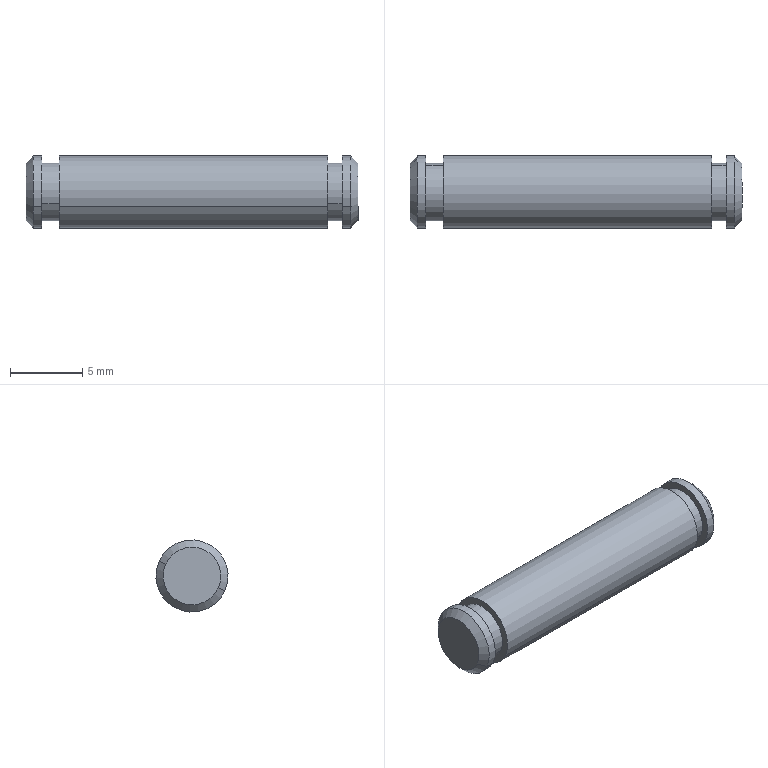Component | SolidWorks | LeverHydraulicRod22-1_HLKA-22_-2-1 | 1 solid | 20 faces | box 23 x 5 x 5 mm | volume 432 mm3 | cylinder 10 | plane 6 | cone 4 | commonest cylinder face diameters 5 x6 4 x4
STEP:
#1=CARTESIAN_POINT('',(-3.072,4.4,-3.091));
#2=VERTEX_POINT('',#1);
#3=CARTESIAN_POINT('',(-3.072,4.58,-3.011));
#4=VERTEX_POINT('',#3);
#5=CARTESIAN_POINT('',(-3.072,4.49,-3.051));
#6=DIRECTION('',(1.,0.,0.));
#7=DIRECTION('',(0.,0.9136,0.4066));
#8=AXIS2_PLACEMENT_3D('',#5,#6,#7);
#9=CIRCLE('',#8,0.09843);
#10=EDGE_CURVE('',#2,#4,#9,.T.);
#11=ORIENTED_EDGE('',*,*,#10,.F.);
#12=CARTESIAN_POINT('',(-3.095,4.4,-3.091));
#13=VERTEX_POINT('',#12);
#14=CARTESIAN_POINT('',(-2.209,4.4,-3.091));
#15=DIRECTION('',(-1.,-0.,-0.));
#16=VECTOR('',#15,39.37);
#17=LINE('',#14,#16);
#18=EDGE_CURVE('',#2,#13,#17,.T.);
#19=ORIENTED_EDGE('',*,*,#18,.T.);
#20=CARTESIAN_POINT('',(-3.095,4.58,-3.011));
#21=VERTEX_POINT('',#20);
#22=CARTESIAN_POINT('',(-3.095,4.49,-3.051));
#23=DIRECTION('',(1.,0.,0.));
#24=DIRECTION('',(0.,-0.9136,-0.4066));
#25=AXIS2_PLACEMENT_3D('',#22,#23,#24);
#26=CIRCLE('',#25,0.09843);
#27=EDGE_CURVE('',#13,#21,#26,.T.);
#28=ORIENTED_EDGE('',*,*,#27,.T.);
#29=CARTESIAN_POINT('',(-2.209,4.58,-3.011));
#30=DIRECTION('',(-1.,-0.,-0.));
#31=VECTOR('',#30,39.37);
#32=LINE('',#29,#31);
#33=EDGE_CURVE('',#4,#21,#32,.T.);
#34=ORIENTED_EDGE('',*,*,#33,.F.);
#35=EDGE_LOOP('',(#11,#19,#28,#34));
#36=FACE_OUTER_BOUND('',#35,.T.);
#37=CARTESIAN_POINT('',(-2.209,4.49,-3.051));
#38=DIRECTION('',(-1.,-0.,-0.));
#39=DIRECTION('',(0.,0.9136,0.4066));
#40=AXIS2_PLACEMENT_3D('',#37,#38,#39);
#41=CYLINDRICAL_SURFACE('',#40,0.09843);
#42=ADVANCED_FACE('',(#36),#41,.T.);
#43=CARTESIAN_POINT('',(-3.115,4.562,-3.019));
#44=VERTEX_POINT('',#43);
#45=CARTESIAN_POINT('',(-3.115,4.418,-3.083));
#46=VERTEX_POINT('',#45);
#47=CARTESIAN_POINT('',(-3.115,4.49,-3.051));
#48=DIRECTION('',(-1.,-0.,-0.));
#49=DIRECTION('',(0.,-0.9136,-0.4066));
#50=AXIS2_PLACEMENT_3D('',#47,#48,#49);
#51=CIRCLE('',#50,0.07874);
#52=EDGE_CURVE('',#44,#46,#51,.T.);
#53=ORIENTED_EDGE('',*,*,#52,.F.);
#54=CARTESIAN_POINT('',(-3.095,4.58,-3.011));
#55=DIRECTION('',(0.7071,0.646,0.2875));
#56=VECTOR('',#55,39.37);
#57=LINE('',#54,#56);
#58=EDGE_CURVE('',#44,#21,#57,.T.);
#59=ORIENTED_EDGE('',*,*,#58,.T.);
#60=ORIENTED_EDGE('',*,*,#27,.F.);
#61=CARTESIAN_POINT('',(-3.095,4.4,-3.091));
#62=DIRECTION('',(0.7071,-0.646,-0.2875));
#63=VECTOR('',#62,39.37);
#64=LINE('',#61,#63);
#65=EDGE_CURVE('',#46,#13,#64,.T.);
#66=ORIENTED_EDGE('',*,*,#65,.F.);
#67=EDGE_LOOP('',(#53,#59,#60,#66));
#68=FACE_OUTER_BOUND('',#67,.T.);
#69=CARTESIAN_POINT('',(-3.095,4.49,-3.051));
#70=DIRECTION('',(1.,0.,0.));
#71=DIRECTION('',(0.,-0.9136,-0.4066));
#72=AXIS2_PLACEMENT_3D('',#69,#70,#71);
#73=CONICAL_SURFACE('',#72,0.09843,0.7854);
#74=ADVANCED_FACE('',(#68),#73,.T.);
#75=CARTESIAN_POINT('',(-2.229,4.58,-3.011));
#76=VERTEX_POINT('',#75);
#77=CARTESIAN_POINT('',(-2.229,4.4,-3.091));
#78=VERTEX_POINT('',#77);
#79=CARTESIAN_POINT('',(-2.229,4.49,-3.051));
#80=DIRECTION('',(-1.,-0.,-0.));
#81=DIRECTION('',(0.,-0.9136,-0.4066));
#82=AXIS2_PLACEMENT_3D('',#79,#80,#81);
#83=CIRCLE('',#82,0.09843);
#84=EDGE_CURVE('',#76,#78,#83,.T.);
#85=ORIENTED_EDGE('',*,*,#84,.T.);
#86=CARTESIAN_POINT('',(-2.253,4.4,-3.091));
#87=VERTEX_POINT('',#86);
#88=CARTESIAN_POINT('',(-2.209,4.4,-3.091));
#89=DIRECTION('',(-1.,-0.,-0.));
#90=VECTOR('',#89,39.37);
#91=LINE('',#88,#90);
#92=EDGE_CURVE('',#78,#87,#91,.T.);
#93=ORIENTED_EDGE('',*,*,#92,.T.);
#94=CARTESIAN_POINT('',(-2.253,4.58,-3.011));
#95=VERTEX_POINT('',#94);
#96=CARTESIAN_POINT('',(-2.253,4.49,-3.051));
#97=DIRECTION('',(1.,0.,0.));
#98=DIRECTION('',(0.,-0.9136,-0.4066));
#99=AXIS2_PLACEMENT_3D('',#96,#97,#98);
#100=CIRCLE('',#99,0.09843);
#101=EDGE_CURVE('',#87,#95,#100,.T.);
#102=ORIENTED_EDGE('',*,*,#101,.T.);
#103=CARTESIAN_POINT('',(-2.209,4.58,-3.011));
#104=DIRECTION('',(-1.,-0.,-0.));
#105=VECTOR('',#104,39.37);
#106=LINE('',#103,#105);
#107=EDGE_CURVE('',#76,#95,#106,.T.);
#108=ORIENTED_EDGE('',*,*,#107,.F.);
#109=EDGE_LOOP('',(#85,#93,#102,#108));
#110=FACE_OUTER_BOUND('',#109,.T.);
#111=CARTESIAN_POINT('',(-2.209,4.49,-3.051));
#112=DIRECTION('',(-1.,-0.,-0.));
#113=DIRECTION('',(0.,0.9136,0.4066));
#114=AXIS2_PLACEMENT_3D('',#111,#112,#113);
#115=CYLINDRICAL_SURFACE('',#114,0.09843);
#116=ADVANCED_FACE('',(#110),#115,.T.);
#117=CARTESIAN_POINT('',(-2.209,4.418,-3.083));
#118=VERTEX_POINT('',#117);
#119=CARTESIAN_POINT('',(-2.209,4.562,-3.019));
#120=VERTEX_POINT('',#119);
#121=CARTESIAN_POINT('',(-2.209,4.49,-3.051));
#122=DIRECTION('',(1.,0.,0.));
#123=DIRECTION('',(0.,-0.9136,-0.4066));
#124=AXIS2_PLACEMENT_3D('',#121,#122,#123);
#125=CIRCLE('',#124,0.07874);
#126=EDGE_CURVE('',#118,#120,#125,.T.);
#127=ORIENTED_EDGE('',*,*,#126,.F.);
#128=CARTESIAN_POINT('',(-2.209,4.418,-3.083));
#129=DIRECTION('',(-0.7071,-0.646,-0.2875));
#130=VECTOR('',#129,39.37);
#131=LINE('',#128,#130);
#132=EDGE_CURVE('',#118,#78,#131,.T.);
#133=ORIENTED_EDGE('',*,*,#132,.T.);
#134=ORIENTED_EDGE('',*,*,#84,.F.);
#135=CARTESIAN_POINT('',(-2.209,4.562,-3.019));
#136=DIRECTION('',(-0.7071,0.646,0.2875));
#137=VECTOR('',#136,39.37);
#138=LINE('',#135,#137);
#139=EDGE_CURVE('',#120,#76,#138,.T.);
#140=ORIENTED_EDGE('',*,*,#139,.F.);
#141=EDGE_LOOP('',(#127,#133,#134,#140));
#142=FACE_OUTER_BOUND('',#141,.T.);
#143=CARTESIAN_POINT('',(-2.209,4.49,-3.051));
#144=DIRECTION('',(-1.,-0.,-0.));
#145=DIRECTION('',(0.,0.9136,0.4066));
#146=AXIS2_PLACEMENT_3D('',#143,#144,#145);
#147=CONICAL_SURFACE('',#146,0.07874,0.7854);
#148=ADVANCED_FACE('',(#142),#147,.T.);
#149=CARTESIAN_POINT('',(-2.253,4.562,-3.019));
#150=VERTEX_POINT('',#149);
#151=CARTESIAN_POINT('',(-2.253,4.418,-3.083));
#152=VERTEX_POINT('',#151);
#153=CARTESIAN_POINT('',(-2.253,4.49,-3.051));
#154=DIRECTION('',(-1.,-0.,-0.));
#155=DIRECTION('',(0.,0.9136,0.4066));
#156=AXIS2_PLACEMENT_3D('',#153,#154,#155);
#157=CIRCLE('',#156,0.07874);
#158=EDGE_CURVE('',#150,#152,#157,.T.);
#159=ORIENTED_EDGE('',*,*,#158,.T.);
#160=CARTESIAN_POINT('',(-2.292,4.418,-3.083));
#161=VERTEX_POINT('',#160);
#162=CARTESIAN_POINT('',(-3.115,4.418,-3.083));
#163=DIRECTION('',(-1.,-0.,-0.));
#164=VECTOR('',#163,39.37);
#165=LINE('',#162,#164);
#166=EDGE_CURVE('',#152,#161,#165,.T.);
#167=ORIENTED_EDGE('',*,*,#166,.T.);
#168=CARTESIAN_POINT('',(-2.292,4.562,-3.019));
#169=VERTEX_POINT('',#168);
#170=CARTESIAN_POINT('',(-2.292,4.49,-3.051));
#171=DIRECTION('',(-1.,-0.,-0.));
#172=DIRECTION('',(0.,0.9136,0.4066));
#173=AXIS2_PLACEMENT_3D('',#170,#171,#172);
#174=CIRCLE('',#173,0.07874);
#175=EDGE_CURVE('',#169,#161,#174,.T.);
#176=ORIENTED_EDGE('',*,*,#175,.F.);
#177=CARTESIAN_POINT('',(-3.115,4.562,-3.019));
#178=DIRECTION('',(-1.,-0.,-0.));
#179=VECTOR('',#178,39.37);
#180=LINE('',#177,#179);
#181=EDGE_CURVE('',#150,#169,#180,.T.);
#182=ORIENTED_EDGE('',*,*,#181,.F.);
#183=EDGE_LOOP('',(#159,#167,#176,#182));
#184=FACE_OUTER_BOUND('',#183,.T.);
#185=CARTESIAN_POINT('',(-3.115,4.49,-3.051));
#186=DIRECTION('',(-1.,-0.,-0.));
#187=DIRECTION('',(0.,0.9136,0.4066));
#188=AXIS2_PLACEMENT_3D('',#185,#186,#187);
#189=CYLINDRICAL_SURFACE('',#188,0.07874);
#190=ADVANCED_FACE('',(#184),#189,.T.);
#191=CARTESIAN_POINT('',(-3.024,4.562,-3.019));
#192=VERTEX_POINT('',#191);
#193=CARTESIAN_POINT('',(-3.024,4.418,-3.083));
#194=VERTEX_POINT('',#193);
#195=CARTESIAN_POINT('',(-3.024,4.49,-3.051));
#196=DIRECTION('',(-1.,-0.,-0.));
#197=DIRECTION('',(0.,0.9136,0.4066));
#198=AXIS2_PLACEMENT_3D('',#195,#196,#197);
#199=CIRCLE('',#198,0.07874);
#200=EDGE_CURVE('',#192,#194,#199,.T.);
#201=ORIENTED_EDGE('',*,*,#200,.T.);
#202=CARTESIAN_POINT('',(-3.072,4.418,-3.083));
#203=VERTEX_POINT('',#202);
#204=CARTESIAN_POINT('',(-3.115,4.418,-3.083));
#205=DIRECTION('',(-1.,-0.,-0.));
#206=VECTOR('',#205,39.37);
#207=LINE('',#204,#206);
#208=EDGE_CURVE('',#194,#203,#207,.T.);
#209=ORIENTED_EDGE('',*,*,#208,.T.);
#210=CARTESIAN_POINT('',(-3.072,4.562,-3.019));
#211=VERTEX_POINT('',#210);
#212=CARTESIAN_POINT('',(-3.072,4.49,-3.051));
#213=DIRECTION('',(-1.,-0.,-0.));
#214=DIRECTION('',(0.,0.9136,0.4066));
#215=AXIS2_PLACEMENT_3D('',#212,#213,#214);
#216=CIRCLE('',#215,0.07874);
#217=EDGE_CURVE('',#211,#203,#216,.T.);
#218=ORIENTED_EDGE('',*,*,#217,.F.);
#219=CARTESIAN_POINT('',(-3.115,4.562,-3.019));
#220=DIRECTION('',(-1.,-0.,-0.));
#221=VECTOR('',#220,39.37);
#222=LINE('',#219,#221);
#223=EDGE_CURVE('',#192,#211,#222,.T.);
#224=ORIENTED_EDGE('',*,*,#223,.F.);
#225=EDGE_LOOP('',(#201,#209,#218,#224));
#226=FACE_OUTER_BOUND('',#225,.T.);
#227=CARTESIAN_POINT('',(-3.115,4.49,-3.051));
#228=DIRECTION('',(-1.,-0.,-0.));
#229=DIRECTION('',(0.,0.9136,0.4066));
#230=AXIS2_PLACEMENT_3D('',#227,#228,#229);
#231=CYLINDRICAL_SURFACE('',#230,0.07874);
#232=ADVANCED_FACE('',(#226),#231,.T.);
#233=CARTESIAN_POINT('',(-2.292,4.58,-3.011));
#234=VERTEX_POINT('',#233);
#235=CARTESIAN_POINT('',(-2.292,4.4,-3.091));
#236=VERTEX_POINT('',#235);
#237=CARTESIAN_POINT('',(-2.292,4.49,-3.051));
#238=DIRECTION('',(-1.,-0.,-0.));
#239=DIRECTION('',(0.,0.9136,0.4066));
#240=AXIS2_PLACEMENT_3D('',#237,#238,#239);
#241=CIRCLE('',#240,0.09843);
#242=EDGE_CURVE('',#234,#236,#241,.T.);
#243=ORIENTED_EDGE('',*,*,#242,.T.);
#244=CARTESIAN_POINT('',(-3.024,4.4,-3.091));
#245=VERTEX_POINT('',#244);
#246=CARTESIAN_POINT('',(-2.209,4.4,-3.091));
#247=DIRECTION('',(-1.,-0.,-0.));
#248=VECTOR('',#247,39.37);
#249=LINE('',#246,#248);
#250=EDGE_CURVE('',#236,#245,#249,.T.);
#251=ORIENTED_EDGE('',*,*,#250,.T.);
#252=CARTESIAN_POINT('',(-3.024,4.58,-3.011));
#253=VERTEX_POINT('',#252);
#254=CARTESIAN_POINT('',(-3.024,4.49,-3.051));
#255=DIRECTION('',(1.,0.,0.));
#256=DIRECTION('',(0.,-0.9136,-0.4066));
#257=AXIS2_PLACEMENT_3D('',#254,#255,#256);
#258=CIRCLE('',#257,0.09843);
#259=EDGE_CURVE('',#245,#253,#258,.T.);
#260=ORIENTED_EDGE('',*,*,#259,.T.);
#261=CARTESIAN_POINT('',(-2.209,4.58,-3.011));
#262=DIRECTION('',(-1.,-0.,-0.));
#263=VECTOR('',#262,39.37);
#264=LINE('',#261,#263);
#265=EDGE_CURVE('',#234,#253,#264,.T.);
#266=ORIENTED_EDGE('',*,*,#265,.F.);
#267=EDGE_LOOP('',(#243,#251,#260,#266));
#268=FACE_OUTER_BOUND('',#267,.T.);
#269=CARTESIAN_POINT('',(-2.209,4.49,-3.051));
#270=DIRECTION('',(-1.,-0.,-0.));
#271=DIRECTION('',(0.,0.9136,0.4066));
#272=AXIS2_PLACEMENT_3D('',#269,#270,#271);
#273=CYLINDRICAL_SURFACE('',#272,0.09843);
#274=ADVANCED_FACE('',(#268),#273,.T.);
#275=CARTESIAN_POINT('',(-2.209,4.49,-3.051));
#276=DIRECTION('',(1.,0.,0.));
#277=DIRECTION('',(0.,-0.9136,-0.4066));
#278=AXIS2_PLACEMENT_3D('',#275,#276,#277);
#279=CIRCLE('',#278,0.07874);
#280=EDGE_CURVE('',#120,#118,#279,.T.);
#281=ORIENTED_EDGE('',*,*,#280,.T.);
#282=ORIENTED_EDGE('',*,*,#126,.T.);
#283=EDGE_LOOP('',(#281,#282));
#284=FACE_OUTER_BOUND('',#283,.T.);
#285=CARTESIAN_POINT('',(-2.209,4.49,-3.051));
#286=DIRECTION('',(1.,0.,0.));
#287=DIRECTION('',(0.,-0.9136,-0.4066));
#288=AXIS2_PLACEMENT_3D('',#285,#286,#287);
#289=PLANE('',#288);
#290=ADVANCED_FACE('',(#284),#289,.T.);
#291=ORIENTED_EDGE('',*,*,#175,.T.);
#292=CARTESIAN_POINT('',(-2.292,4.49,-3.051));
#293=DIRECTION('',(-1.,-0.,-0.));
#294=DIRECTION('',(0.,0.9136,0.4066));
#295=AXIS2_PLACEMENT_3D('',#292,#293,#294);
#296=CIRCLE('',#295,0.07874);
#297=EDGE_CURVE('',#161,#169,#296,.T.);
#298=ORIENTED_EDGE('',*,*,#297,.T.);
#299=EDGE_LOOP('',(#291,#298));
#300=FACE_BOUND('',#299,.T.);
#301=ORIENTED_EDGE('',*,*,#242,.F.);
#302=CARTESIAN_POINT('',(-2.292,4.49,-3.051));
#303=DIRECTION('',(-1.,-0.,-0.));
#304=DIRECTION('',(0.,0.9136,0.4066));
#305=AXIS2_PLACEMENT_3D('',#302,#303,#304);
#306=CIRCLE('',#305,0.09843);
#307=EDGE_CURVE('',#236,#234,#306,.T.);
#308=ORIENTED_EDGE('',*,*,#307,.F.);
#309=EDGE_LOOP('',(#301,#308));
#310=FACE_OUTER_BOUND('',#309,.T.);
#311=CARTESIAN_POINT('',(-2.292,4.621,-2.993));
#312=DIRECTION('',(-1.,0.,-0.));
#313=DIRECTION('',(-0.,-0.4066,0.9136));
#314=AXIS2_PLACEMENT_3D('',#311,#312,#313);
#315=PLANE('',#314);
#316=ADVANCED_FACE('',(#300,#310),#315,.F.);
#317=ORIENTED_EDGE('',*,*,#158,.F.);
#318=CARTESIAN_POINT('',(-2.253,4.49,-3.051));
#319=DIRECTION('',(-1.,-0.,-0.));
#320=DIRECTION('',(0.,0.9136,0.4066));
#321=AXIS2_PLACEMENT_3D('',#318,#319,#320);
#322=CIRCLE('',#321,0.07874);
#323=EDGE_CURVE('',#152,#150,#322,.T.);
#324=ORIENTED_EDGE('',*,*,#323,.F.);
#325=EDGE_LOOP('',(#317,#324));
#326=FACE_BOUND('',#325,.T.);
#327=CARTESIAN_POINT('',(-2.253,4.49,-3.051));
#328=DIRECTION('',(1.,0.,0.));
#329=DIRECTION('',(0.,-0.9136,-0.4066));
#330=AXIS2_PLACEMENT_3D('',#327,#328,#329);
#331=CIRCLE('',#330,0.09843);
#332=EDGE_CURVE('',#95,#87,#331,.T.);
#333=ORIENTED_EDGE('',*,*,#332,.F.);
#334=ORIENTED_EDGE('',*,*,#101,.F.);
#335=EDGE_LOOP('',(#333,#334));
#336=FACE_OUTER_BOUND('',#335,.T.);
#337=CARTESIAN_POINT('',(-2.253,4.621,-2.993));
#338=DIRECTION('',(1.,0.,0.));
#339=DIRECTION('',(0.,-0.9136,-0.4066));
#340=AXIS2_PLACEMENT_3D('',#337,#338,#339);
#341=PLANE('',#340);
#342=ADVANCED_FACE('',(#326,#336),#341,.F.);
#343=ORIENTED_EDGE('',*,*,#200,.F.);
#344=CARTESIAN_POINT('',(-3.024,4.49,-3.051));
#345=DIRECTION('',(-1.,-0.,-0.));
#346=DIRECTION('',(0.,0.9136,0.4066));
#347=AXIS2_PLACEMENT_3D('',#344,#345,#346);
#348=CIRCLE('',#347,0.07874);
#349=EDGE_CURVE('',#194,#192,#348,.T.);
#350=ORIENTED_EDGE('',*,*,#349,.F.);
#351=EDGE_LOOP('',(#343,#350));
#352=FACE_BOUND('',#351,.T.);
#353=CARTESIAN_POINT('',(-3.024,4.49,-3.051));
#354=DIRECTION('',(1.,0.,0.));
#355=DIRECTION('',(0.,-0.9136,-0.4066));
#356=AXIS2_PLACEMENT_3D('',#353,#354,#355);
#357=CIRCLE('',#356,0.09843);
#358=EDGE_CURVE('',#253,#245,#357,.T.);
#359=ORIENTED_EDGE('',*,*,#358,.F.);
#360=ORIENTED_EDGE('',*,*,#259,.F.);
#361=EDGE_LOOP('',(#359,#360));
#362=FACE_OUTER_BOUND('',#361,.T.);
#363=CARTESIAN_POINT('',(-3.024,4.596,-3.004));
#364=DIRECTION('',(1.,0.,0.));
#365=DIRECTION('',(0.,-0.9136,-0.4066));
#366=AXIS2_PLACEMENT_3D('',#363,#364,#365);
#367=PLANE('',#366);
#368=ADVANCED_FACE('',(#352,#362),#367,.F.);
#369=ORIENTED_EDGE('',*,*,#250,.F.);
#370=ORIENTED_EDGE('',*,*,#307,.T.);
#371=ORIENTED_EDGE('',*,*,#265,.T.);
#372=ORIENTED_EDGE('',*,*,#358,.T.);
#373=EDGE_LOOP('',(#369,#370,#371,#372));
#374=FACE_OUTER_BOUND('',#373,.T.);
#375=CARTESIAN_POINT('',(-2.209,4.49,-3.051));
#376=DIRECTION('',(-1.,-0.,-0.));
#377=DIRECTION('',(0.,0.9136,0.4066));
#378=AXIS2_PLACEMENT_3D('',#375,#376,#377);
#379=CYLINDRICAL_SURFACE('',#378,0.09843);
#380=ADVANCED_FACE('',(#374),#379,.T.);
#381=ORIENTED_EDGE('',*,*,#208,.F.);
#382=ORIENTED_EDGE('',*,*,#349,.T.);
#383=ORIENTED_EDGE('',*,*,#223,.T.);
#384=CARTESIAN_POINT('',(-3.072,4.49,-3.051));
#385=DIRECTION('',(-1.,-0.,-0.));
#386=DIRECTION('',(0.,0.9136,0.4066));
#387=AXIS2_PLACEMENT_3D('',#384,#385,#386);
#388=CIRCLE('',#387,0.07874);
#389=EDGE_CURVE('',#203,#211,#388,.T.);
#390=ORIENTED_EDGE('',*,*,#389,.F.);
#391=EDGE_LOOP('',(#381,#382,#383,#390));
#392=FACE_OUTER_BOUND('',#391,.T.);
#393=CARTESIAN_POINT('',(-3.115,4.49,-3.051));
#394=DIRECTION('',(-1.,-0.,-0.));
#395=DIRECTION('',(0.,0.9136,0.4066));
#396=AXIS2_PLACEMENT_3D('',#393,#394,#395);
#397=CYLINDRICAL_SURFACE('',#396,0.07874);
#398=ADVANCED_FACE('',(#392),#397,.T.);
#399=ORIENTED_EDGE('',*,*,#166,.F.);
#400=ORIENTED_EDGE('',*,*,#323,.T.);
#401=ORIENTED_EDGE('',*,*,#181,.T.);
#402=ORIENTED_EDGE('',*,*,#297,.F.);
#403=EDGE_LOOP('',(#399,#400,#401,#402));
#404=FACE_OUTER_BOUND('',#403,.T.);
#405=CARTESIAN_POINT('',(-3.115,4.49,-3.051));
#406=DIRECTION('',(-1.,-0.,-0.));
#407=DIRECTION('',(0.,0.9136,0.4066));
#408=AXIS2_PLACEMENT_3D('',#405,#406,#407);
#409=CYLINDRICAL_SURFACE('',#408,0.07874);
#410=ADVANCED_FACE('',(#404),#409,.T.);
#411=ORIENTED_EDGE('',*,*,#132,.F.);
#412=ORIENTED_EDGE('',*,*,#280,.F.);
#413=ORIENTED_EDGE('',*,*,#139,.T.);
#414=CARTESIAN_POINT('',(-2.229,4.49,-3.051));
#415=DIRECTION('',(-1.,-0.,-0.));
#416=DIRECTION('',(0.,-0.9136,-0.4066));
#417=AXIS2_PLACEMENT_3D('',#414,#415,#416);
#418=CIRCLE('',#417,0.09843);
#419=EDGE_CURVE('',#78,#76,#418,.T.);
#420=ORIENTED_EDGE('',*,*,#419,.F.);
#421=EDGE_LOOP('',(#411,#412,#413,#420));
#422=FACE_OUTER_BOUND('',#421,.T.);
#423=CARTESIAN_POINT('',(-2.209,4.49,-3.051));
#424=DIRECTION('',(-1.,-0.,-0.));
#425=DIRECTION('',(0.,0.9136,0.4066));
#426=AXIS2_PLACEMENT_3D('',#423,#424,#425);
#427=CONICAL_SURFACE('',#426,0.07874,0.7854);
#428=ADVANCED_FACE('',(#422),#427,.T.);
#429=ORIENTED_EDGE('',*,*,#92,.F.);
#430=ORIENTED_EDGE('',*,*,#419,.T.);
#431=ORIENTED_EDGE('',*,*,#107,.T.);
#432=ORIENTED_EDGE('',*,*,#332,.T.);
#433=EDGE_LOOP('',(#429,#430,#431,#432));
#434=FACE_OUTER_BOUND('',#433,.T.);
#435=CARTESIAN_POINT('',(-2.209,4.49,-3.051));
#436=DIRECTION('',(-1.,-0.,-0.));
#437=DIRECTION('',(0.,0.9136,0.4066));
#438=AXIS2_PLACEMENT_3D('',#435,#436,#437);
#439=CYLINDRICAL_SURFACE('',#438,0.09843);
#440=ADVANCED_FACE('',(#434),#439,.T.);
#441=CARTESIAN_POINT('',(-3.072,4.49,-3.051));
#442=DIRECTION('',(1.,0.,0.));
#443=DIRECTION('',(0.,0.9136,0.4066));
#444=AXIS2_PLACEMENT_3D('',#441,#442,#443);
#445=CIRCLE('',#444,0.09843);
#446=EDGE_CURVE('',#4,#2,#445,.T.);
#447=ORIENTED_EDGE('',*,*,#446,.T.);
#448=ORIENTED_EDGE('',*,*,#10,.T.);
#449=EDGE_LOOP('',(#447,#448));
#450=FACE_OUTER_BOUND('',#449,.T.);
#451=ORIENTED_EDGE('',*,*,#217,.T.);
#452=ORIENTED_EDGE('',*,*,#389,.T.);
#453=EDGE_LOOP('',(#451,#452));
#454=FACE_BOUND('',#453,.T.);
#455=CARTESIAN_POINT('',(-3.072,4.538,-3.159));
#456=DIRECTION('',(-1.,-0.,-0.));
#457=DIRECTION('',(-0.,0.9136,0.4066));
#458=AXIS2_PLACEMENT_3D('',#455,#456,#457);
#459=PLANE('',#458);
#460=ADVANCED_FACE('',(#450,#454),#459,.F.);
#461=CARTESIAN_POINT('',(-3.115,4.49,-3.051));
#462=DIRECTION('',(-1.,-0.,-0.));
#463=DIRECTION('',(0.,-0.9136,-0.4066));
#464=AXIS2_PLACEMENT_3D('',#461,#462,#463);
#465=CIRCLE('',#464,0.07874);
#466=EDGE_CURVE('',#46,#44,#465,.T.);
#467=ORIENTED_EDGE('',*,*,#466,.T.);
#468=ORIENTED_EDGE('',*,*,#52,.T.);
#469=EDGE_LOOP('',(#467,#468));
#470=FACE_OUTER_BOUND('',#469,.T.);
#471=CARTESIAN_POINT('',(-3.115,4.49,-3.051));
#472=DIRECTION('',(1.,0.,0.));
#473=DIRECTION('',(0.,-0.9136,-0.4066));
#474=AXIS2_PLACEMENT_3D('',#471,#472,#473);
#475=PLANE('',#474);
#476=ADVANCED_FACE('',(#470),#475,.F.);
#477=ORIENTED_EDGE('',*,*,#58,.F.);
#478=ORIENTED_EDGE('',*,*,#466,.F.);
#479=ORIENTED_EDGE('',*,*,#65,.T.);
#480=CARTESIAN_POINT('',(-3.095,4.49,-3.051));
#481=DIRECTION('',(1.,0.,0.));
#482=DIRECTION('',(0.,-0.9136,-0.4066));
#483=AXIS2_PLACEMENT_3D('',#480,#481,#482);
#484=CIRCLE('',#483,0.09843);
#485=EDGE_CURVE('',#21,#13,#484,.T.);
#486=ORIENTED_EDGE('',*,*,#485,.F.);
#487=EDGE_LOOP('',(#477,#478,#479,#486));
#488=FACE_OUTER_BOUND('',#487,.T.);
#489=CARTESIAN_POINT('',(-3.095,4.49,-3.051));
#490=DIRECTION('',(1.,0.,0.));
#491=DIRECTION('',(0.,-0.9136,-0.4066));
#492=AXIS2_PLACEMENT_3D('',#489,#490,#491);
#493=CONICAL_SURFACE('',#492,0.09843,0.7854);
#494=ADVANCED_FACE('',(#488),#493,.T.);
#495=ORIENTED_EDGE('',*,*,#18,.F.);
#496=ORIENTED_EDGE('',*,*,#446,.F.);
#497=ORIENTED_EDGE('',*,*,#33,.T.);
#498=ORIENTED_EDGE('',*,*,#485,.T.);
#499=EDGE_LOOP('',(#495,#496,#497,#498));
#500=FACE_OUTER_BOUND('',#499,.T.);
#501=CARTESIAN_POINT('',(-2.209,4.49,-3.051));
#502=DIRECTION('',(-1.,-0.,-0.));
#503=DIRECTION('',(0.,0.9136,0.4066));
#504=AXIS2_PLACEMENT_3D('',#501,#502,#503);
#505=CYLINDRICAL_SURFACE('',#504,0.09843);
#506=ADVANCED_FACE('',(#500),#505,.T.);
#507=CLOSED_SHELL('',(#42,#74,#116,#148,#190,#232,#274,#290,#316,#342,#368,#380,#398,#410,#428,#440,#460,#476,#494,#506));
#508=MANIFOLD_SOLID_BREP('',#507);
#509=CARTESIAN_POINT('',(0.,0.,0.));
#510=DIRECTION('',(0.,0.,1.));
#511=DIRECTION('',(1.,0.,0.));
#512=AXIS2_PLACEMENT_3D('',#509,#510,#511);
#513=(LENGTH_UNIT()NAMED_UNIT(*)SI_UNIT($,.METRE.));
#514=LENGTH_MEASURE_WITH_UNIT(LENGTH_MEASURE(0.0254),#513);
#515=DIMENSIONAL_EXPONENTS(1.,0.,0.,0.,0.,0.,0.);
#516=(CONVERSION_BASED_UNIT('',#514)LENGTH_UNIT()NAMED_UNIT(#515));
#517=UNCERTAINTY_MEASURE_WITH_UNIT(LENGTH_MEASURE(0.00001),#516,'','');
#518=(NAMED_UNIT(*)PLANE_ANGLE_UNIT()SI_UNIT($,.RADIAN.));
#519=(NAMED_UNIT(*)SI_UNIT($,.STERADIAN.)SOLID_ANGLE_UNIT());
#520=(GEOMETRIC_REPRESENTATION_CONTEXT(3)GLOBAL_UNCERTAINTY_ASSIGNED_CONTEXT((#517))GLOBAL_UNIT_ASSIGNED_CONTEXT((#516,#518,#519))REPRESENTATION_CONTEXT('',''));
#521=ADVANCED_BREP_SHAPE_REPRESENTATION('',(#508,#512),#520);
#522=COLOUR_RGB('',0.7922,0.8196,0.9333);
#523=FILL_AREA_STYLE_COLOUR('',#522);
#524=FILL_AREA_STYLE('',(#523));
#525=SURFACE_STYLE_FILL_AREA(#524);
#526=SURFACE_SIDE_STYLE('',(#525));
#527=SURFACE_STYLE_USAGE(.BOTH.,#526);
#528=PRESENTATION_STYLE_ASSIGNMENT((#527));
#529=STYLED_ITEM('',(#528),#508);
#530=(LENGTH_UNIT()NAMED_UNIT(*)SI_UNIT($,.METRE.));
#531=LENGTH_MEASURE_WITH_UNIT(LENGTH_MEASURE(0.0254),#530);
#532=DIMENSIONAL_EXPONENTS(1.,0.,0.,0.,0.,0.,0.);
#533=(CONVERSION_BASED_UNIT('',#531)LENGTH_UNIT()NAMED_UNIT(#532));
#534=UNCERTAINTY_MEASURE_WITH_UNIT(LENGTH_MEASURE(0.00001),#533,'','');
#535=(NAMED_UNIT(*)PLANE_ANGLE_UNIT()SI_UNIT($,.RADIAN.));
#536=(NAMED_UNIT(*)SI_UNIT($,.STERADIAN.)SOLID_ANGLE_UNIT());
#537=(GEOMETRIC_REPRESENTATION_CONTEXT(3)GLOBAL_UNCERTAINTY_ASSIGNED_CONTEXT((#534))GLOBAL_UNIT_ASSIGNED_CONTEXT((#533,#535,#536))REPRESENTATION_CONTEXT('',''));
#538=MECHANICAL_DESIGN_GEOMETRIC_PRESENTATION_REPRESENTATION('',(#529),#537);
#539=PRESENTATION_LAYER_ASSIGNMENT('','',(#529));